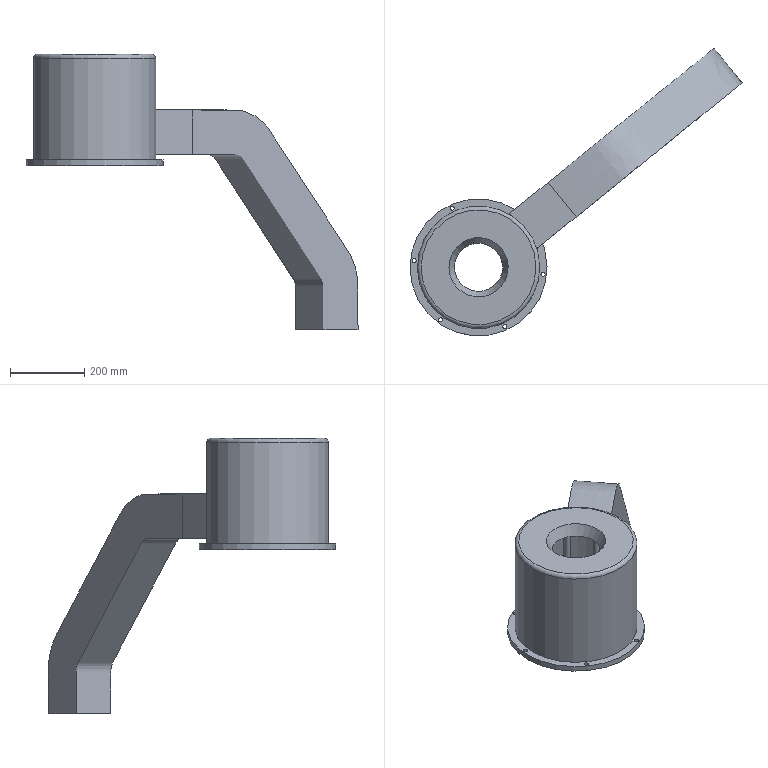Component | NX | STORAGE_BIN | 1 solid | 58 faces | volume 10148047 mm3 | cylinder 33 | plane 17 | spline 6 | cone 1 | torus 1 | commonest cylinder face diameters 310 x13 17 x12 11 x6 370 x1 330 x1